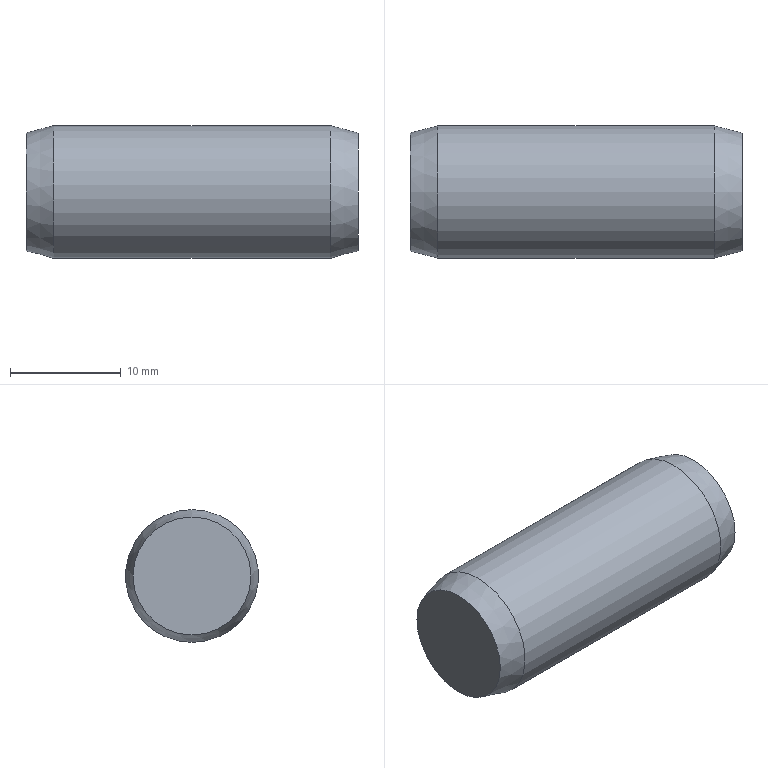Component | NX | GB-T119_1-2000_12X30 | 1 solid | 5 faces | box 30 x 12 x 12 mm | volume 3332 mm3 | plane 2 | cone 2 | cylinder 1 | commonest cylinder face diameters 12 x1
STEP:
#1=CARTESIAN_POINT('',(0.,0.,0.));
#2=DIRECTION('',(0.,0.,1.));
#3=DIRECTION('',(1.,0.,0.));
#4=AXIS2_PLACEMENT_3D('',#1,#2,#3);
#5=CARTESIAN_POINT('',(545.625,-95.909,-26.727));
#6=VERTEX_POINT('',#5);
#7=CARTESIAN_POINT('',(545.625,-95.909,-32.057));
#8=DIRECTION('',(-1.,0.,0.));
#9=DIRECTION('',(0.,0.,1.));
#10=AXIS2_PLACEMENT_3D('',#7,#8,#9);
#11=CIRCLE('',#10,5.33);
#12=CARTESIAN_POINT('',(545.625,-95.909,-32.057));
#13=DIRECTION('',(-1.,0.,0.));
#14=DIRECTION('',(0.,0.,1.));
#15=AXIS2_PLACEMENT_3D('',#12,#13,#14);
#16=PLANE('',#15);
#17=CARTESIAN_POINT('',(0.,0.));
#18=DIRECTION('',(1.,0.));
#19=AXIS2_PLACEMENT_2D('',#17,#18);
#20=CIRCLE('',#19,5.33);
#21=(GEOMETRIC_REPRESENTATION_CONTEXT(2)PARAMETRIC_REPRESENTATION_CONTEXT()REPRESENTATION_CONTEXT('',''));
#22=DEFINITIONAL_REPRESENTATION('',(#20),#21);
#23=PCURVE('',#16,#22);
#24=CARTESIAN_POINT('',(545.625,-95.909,-32.057));
#25=DIRECTION('',(1.,0.,0.));
#26=DIRECTION('',(0.,0.,-1.));
#27=AXIS2_PLACEMENT_3D('',#24,#25,#26);
#28=CONICAL_SURFACE('',#27,5.33,0.2618);
#29=CARTESIAN_POINT('',(9.425,-0.));
#30=DIRECTION('',(-1.,0.));
#31=VECTOR('',#30,1.);
#32=LINE('',#29,#31);
#33=(GEOMETRIC_REPRESENTATION_CONTEXT(2)PARAMETRIC_REPRESENTATION_CONTEXT()REPRESENTATION_CONTEXT('',''));
#34=DEFINITIONAL_REPRESENTATION('',(#32),#33);
#35=PCURVE('',#28,#34);
#36=SURFACE_CURVE('',#11,(#23,#35),.PCURVE_S1.);
#37=EDGE_CURVE('',#6,#6,#36,.T.);
#38=ORIENTED_EDGE('',*,*,#37,.T.);
#39=EDGE_LOOP('',(#38));
#40=FACE_BOUND('',#39,.T.);
#41=ADVANCED_FACE('',(#40),#16,.T.);
#42=CARTESIAN_POINT('',(548.125,-95.909,-26.057));
#43=VERTEX_POINT('',#42);
#44=CARTESIAN_POINT('',(548.125,-95.909,-32.057));
#45=DIRECTION('',(-1.,0.,0.));
#46=DIRECTION('',(0.,0.,1.));
#47=AXIS2_PLACEMENT_3D('',#44,#45,#46);
#48=CIRCLE('',#47,6.);
#49=CARTESIAN_POINT('',(9.425,2.5));
#50=DIRECTION('',(-1.,0.));
#51=VECTOR('',#50,1.);
#52=LINE('',#49,#51);
#53=(GEOMETRIC_REPRESENTATION_CONTEXT(2)PARAMETRIC_REPRESENTATION_CONTEXT()REPRESENTATION_CONTEXT('',''));
#54=DEFINITIONAL_REPRESENTATION('',(#52),#53);
#55=PCURVE('',#28,#54);
#56=CARTESIAN_POINT('',(575.625,-95.909,-32.057));
#57=DIRECTION('',(-1.,0.,0.));
#58=DIRECTION('',(0.,0.,1.));
#59=AXIS2_PLACEMENT_3D('',#56,#57,#58);
#60=CYLINDRICAL_SURFACE('',#59,6.);
#61=CARTESIAN_POINT('',(0.,27.5));
#62=DIRECTION('',(1.,0.));
#63=VECTOR('',#62,1.);
#64=LINE('',#61,#63);
#65=(GEOMETRIC_REPRESENTATION_CONTEXT(2)PARAMETRIC_REPRESENTATION_CONTEXT()REPRESENTATION_CONTEXT('',''));
#66=DEFINITIONAL_REPRESENTATION('',(#64),#65);
#67=PCURVE('',#60,#66);
#68=SURFACE_CURVE('',#48,(#55,#67),.PCURVE_S1.);
#69=EDGE_CURVE('',#43,#43,#68,.T.);
#70=ORIENTED_EDGE('',*,*,#69,.T.);
#71=CARTESIAN_POINT('',(545.625,-95.909,-26.727));
#72=CARTESIAN_POINT('',(548.125,-95.909,-26.057));
#73=B_SPLINE_CURVE_WITH_KNOTS('',1,(#71,#72),.UNSPECIFIED.,.F.,.F.,(2,2),(-0.,2.588),.PIECEWISE_BEZIER_KNOTS.);
#74=CARTESIAN_POINT('',(3.142,0.));
#75=DIRECTION('',(0.,1.));
#76=VECTOR('',#75,1.);
#77=LINE('',#74,#76);
#78=(GEOMETRIC_REPRESENTATION_CONTEXT(2)PARAMETRIC_REPRESENTATION_CONTEXT()REPRESENTATION_CONTEXT('',''));
#79=DEFINITIONAL_REPRESENTATION('',(#77),#78);
#80=PCURVE('',#28,#79);
#81=CARTESIAN_POINT('',(9.425,0.));
#82=DIRECTION('',(0.,1.));
#83=VECTOR('',#82,1.);
#84=LINE('',#81,#83);
#85=(GEOMETRIC_REPRESENTATION_CONTEXT(2)PARAMETRIC_REPRESENTATION_CONTEXT()REPRESENTATION_CONTEXT('',''));
#86=DEFINITIONAL_REPRESENTATION('',(#84),#85);
#87=PCURVE('',#28,#86);
#88=SEAM_CURVE('',#73,(#80,#87),.PCURVE_S1.);
#89=EDGE_CURVE('',#6,#43,#88,.T.);
#90=ORIENTED_EDGE('',*,*,#89,.F.);
#91=ORIENTED_EDGE('',*,*,#37,.F.);
#92=ORIENTED_EDGE('',*,*,#89,.T.);
#93=EDGE_LOOP('',(#70,#90,#91,#92));
#94=FACE_BOUND('',#93,.T.);
#95=ADVANCED_FACE('',(#94),#28,.T.);
#96=CARTESIAN_POINT('',(573.125,-95.909,-26.057));
#97=VERTEX_POINT('',#96);
#98=CARTESIAN_POINT('',(573.125,-95.909,-32.057));
#99=DIRECTION('',(-1.,0.,0.));
#100=DIRECTION('',(0.,0.,1.));
#101=AXIS2_PLACEMENT_3D('',#98,#99,#100);
#102=CIRCLE('',#101,6.);
#103=CARTESIAN_POINT('',(0.,2.5));
#104=DIRECTION('',(1.,0.));
#105=VECTOR('',#104,1.);
#106=LINE('',#103,#105);
#107=(GEOMETRIC_REPRESENTATION_CONTEXT(2)PARAMETRIC_REPRESENTATION_CONTEXT()REPRESENTATION_CONTEXT('',''));
#108=DEFINITIONAL_REPRESENTATION('',(#106),#107);
#109=PCURVE('',#60,#108);
#110=CARTESIAN_POINT('',(573.125,-95.909,-32.057));
#111=DIRECTION('',(-1.,0.,0.));
#112=DIRECTION('',(0.,0.,1.));
#113=AXIS2_PLACEMENT_3D('',#110,#111,#112);
#114=CONICAL_SURFACE('',#113,6.,0.2618);
#115=CARTESIAN_POINT('',(0.,0.));
#116=DIRECTION('',(1.,0.));
#117=VECTOR('',#116,1.);
#118=LINE('',#115,#117);
#119=(GEOMETRIC_REPRESENTATION_CONTEXT(2)PARAMETRIC_REPRESENTATION_CONTEXT()REPRESENTATION_CONTEXT('',''));
#120=DEFINITIONAL_REPRESENTATION('',(#118),#119);
#121=PCURVE('',#114,#120);
#122=SURFACE_CURVE('',#102,(#109,#121),.PCURVE_S1.);
#123=EDGE_CURVE('',#97,#97,#122,.T.);
#124=ORIENTED_EDGE('',*,*,#123,.T.);
#125=CARTESIAN_POINT('',(573.125,-95.909,-26.057));
#126=CARTESIAN_POINT('',(548.125,-95.909,-26.057));
#127=B_SPLINE_CURVE_WITH_KNOTS('',1,(#125,#126),.UNSPECIFIED.,.F.,.F.,(2,2),(2.5,27.5),.PIECEWISE_BEZIER_KNOTS.);
#128=CARTESIAN_POINT('',(6.283,0.));
#129=DIRECTION('',(0.,1.));
#130=VECTOR('',#129,1.);
#131=LINE('',#128,#130);
#132=(GEOMETRIC_REPRESENTATION_CONTEXT(2)PARAMETRIC_REPRESENTATION_CONTEXT()REPRESENTATION_CONTEXT('',''));
#133=DEFINITIONAL_REPRESENTATION('',(#131),#132);
#134=PCURVE('',#60,#133);
#135=CARTESIAN_POINT('',(0.,0.));
#136=DIRECTION('',(0.,1.));
#137=VECTOR('',#136,1.);
#138=LINE('',#135,#137);
#139=(GEOMETRIC_REPRESENTATION_CONTEXT(2)PARAMETRIC_REPRESENTATION_CONTEXT()REPRESENTATION_CONTEXT('',''));
#140=DEFINITIONAL_REPRESENTATION('',(#138),#139);
#141=PCURVE('',#60,#140);
#142=SEAM_CURVE('',#127,(#134,#141),.PCURVE_S1.);
#143=EDGE_CURVE('',#97,#43,#142,.T.);
#144=ORIENTED_EDGE('',*,*,#143,.T.);
#145=ORIENTED_EDGE('',*,*,#69,.F.);
#146=ORIENTED_EDGE('',*,*,#143,.F.);
#147=EDGE_LOOP('',(#124,#144,#145,#146));
#148=FACE_BOUND('',#147,.T.);
#149=ADVANCED_FACE('',(#148),#60,.T.);
#150=CARTESIAN_POINT('',(575.625,-95.909,-26.727));
#151=VERTEX_POINT('',#150);
#152=CARTESIAN_POINT('',(575.625,-95.909,-32.057));
#153=DIRECTION('',(-1.,0.,0.));
#154=DIRECTION('',(0.,0.,1.));
#155=AXIS2_PLACEMENT_3D('',#152,#153,#154);
#156=CIRCLE('',#155,5.33);
#157=CARTESIAN_POINT('',(0.,-2.5));
#158=DIRECTION('',(1.,0.));
#159=VECTOR('',#158,1.);
#160=LINE('',#157,#159);
#161=(GEOMETRIC_REPRESENTATION_CONTEXT(2)PARAMETRIC_REPRESENTATION_CONTEXT()REPRESENTATION_CONTEXT('',''));
#162=DEFINITIONAL_REPRESENTATION('',(#160),#161);
#163=PCURVE('',#114,#162);
#164=CARTESIAN_POINT('',(575.625,-95.909,-37.387));
#165=DIRECTION('',(1.,0.,0.));
#166=DIRECTION('',(0.,0.,-1.));
#167=AXIS2_PLACEMENT_3D('',#164,#165,#166);
#168=PLANE('',#167);
#169=CARTESIAN_POINT('',(-10.66,0.));
#170=CARTESIAN_POINT('',(-10.66,9.232));
#171=CARTESIAN_POINT('',(-2.665,4.616));
#172=CARTESIAN_POINT('',(5.33,0.));
#173=CARTESIAN_POINT('',(-2.665,-4.616));
#174=CARTESIAN_POINT('',(-10.66,-9.232));
#175=CARTESIAN_POINT('',(-10.66,0.));
#176=(BOUNDED_CURVE()B_SPLINE_CURVE(2,(#169,#170,#171,#172,#173,#174,#175),.UNSPECIFIED.,.T.,.F.)B_SPLINE_CURVE_WITH_KNOTS((1,2,2,2,2,1),(-2.094,0.,2.094,4.189,6.283,8.378),.UNSPECIFIED.)CURVE()GEOMETRIC_REPRESENTATION_ITEM()RATIONAL_B_SPLINE_CURVE((1.,0.5,1.,0.5,1.,0.5,1.))REPRESENTATION_ITEM(''));
#177=(GEOMETRIC_REPRESENTATION_CONTEXT(2)PARAMETRIC_REPRESENTATION_CONTEXT()REPRESENTATION_CONTEXT('',''));
#178=DEFINITIONAL_REPRESENTATION('',(#176),#177);
#179=PCURVE('',#168,#178);
#180=SURFACE_CURVE('',#156,(#163,#179),.PCURVE_S1.);
#181=EDGE_CURVE('',#151,#151,#180,.T.);
#182=ORIENTED_EDGE('',*,*,#181,.T.);
#183=CARTESIAN_POINT('',(575.625,-95.909,-26.727));
#184=CARTESIAN_POINT('',(573.125,-95.909,-26.057));
#185=B_SPLINE_CURVE_WITH_KNOTS('',1,(#183,#184),.UNSPECIFIED.,.F.,.F.,(2,2),(-2.588,0.),.PIECEWISE_BEZIER_KNOTS.);
#186=CARTESIAN_POINT('',(6.283,0.));
#187=DIRECTION('',(0.,1.));
#188=VECTOR('',#187,1.);
#189=LINE('',#186,#188);
#190=(GEOMETRIC_REPRESENTATION_CONTEXT(2)PARAMETRIC_REPRESENTATION_CONTEXT()REPRESENTATION_CONTEXT('',''));
#191=DEFINITIONAL_REPRESENTATION('',(#189),#190);
#192=PCURVE('',#114,#191);
#193=CARTESIAN_POINT('',(0.,0.));
#194=DIRECTION('',(0.,1.));
#195=VECTOR('',#194,1.);
#196=LINE('',#193,#195);
#197=(GEOMETRIC_REPRESENTATION_CONTEXT(2)PARAMETRIC_REPRESENTATION_CONTEXT()REPRESENTATION_CONTEXT('',''));
#198=DEFINITIONAL_REPRESENTATION('',(#196),#197);
#199=PCURVE('',#114,#198);
#200=SEAM_CURVE('',#185,(#192,#199),.PCURVE_S1.);
#201=EDGE_CURVE('',#151,#97,#200,.T.);
#202=ORIENTED_EDGE('',*,*,#201,.T.);
#203=ORIENTED_EDGE('',*,*,#123,.F.);
#204=ORIENTED_EDGE('',*,*,#201,.F.);
#205=EDGE_LOOP('',(#182,#202,#203,#204));
#206=FACE_BOUND('',#205,.T.);
#207=ADVANCED_FACE('',(#206),#114,.T.);
#208=ORIENTED_EDGE('',*,*,#181,.F.);
#209=EDGE_LOOP('',(#208));
#210=FACE_BOUND('',#209,.T.);
#211=ADVANCED_FACE('',(#210),#168,.T.);
#212=CLOSED_SHELL('',(#41,#95,#149,#207,#211));
#213=MANIFOLD_SOLID_BREP('',#212);
#214=(LENGTH_UNIT()NAMED_UNIT(*)SI_UNIT(.MILLI.,.METRE.));
#215=UNCERTAINTY_MEASURE_WITH_UNIT(LENGTH_MEASURE(0.00001),#214,'','');
#216=(NAMED_UNIT(*)PLANE_ANGLE_UNIT()SI_UNIT($,.RADIAN.));
#217=(NAMED_UNIT(*)SI_UNIT($,.STERADIAN.)SOLID_ANGLE_UNIT());
#218=(GEOMETRIC_REPRESENTATION_CONTEXT(3)GLOBAL_UNCERTAINTY_ASSIGNED_CONTEXT((#215))GLOBAL_UNIT_ASSIGNED_CONTEXT((#214,#216,#217))REPRESENTATION_CONTEXT('',''));
#219=ADVANCED_BREP_SHAPE_REPRESENTATION('',(#4,#213),#218);